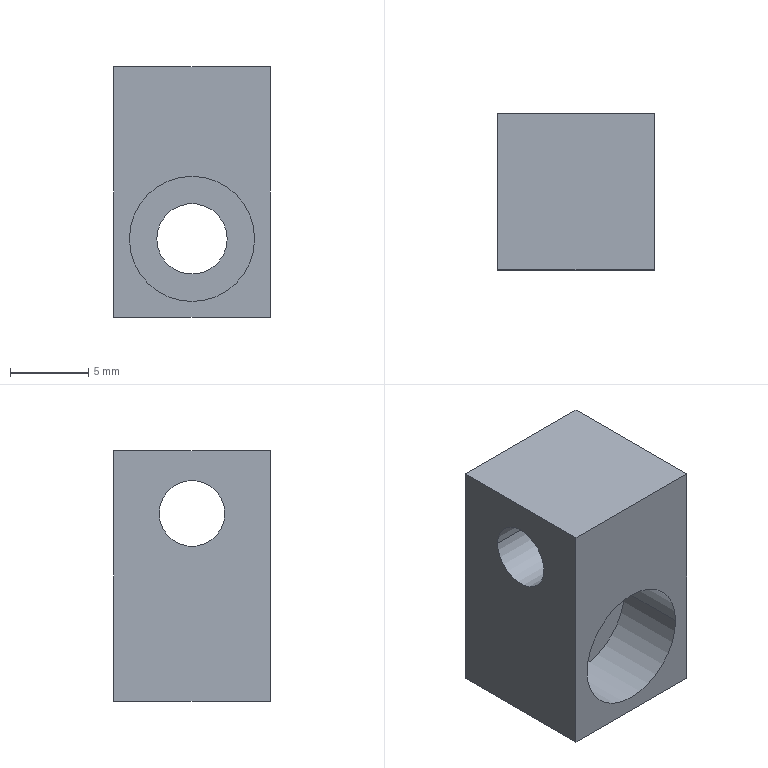Component | SolidWorks | 09HHHHHH8-2 | 1 solid | 13 faces | box 10 x 10 x 16 mm | volume 1144 mm3 | plane 7 | cylinder 6 | commonest cylinder face diameters 4.2 x2 8 x2 4.5 x2
build123d program:
from build123d import *

# Parameters (mm, degrees)
SKETCH1_W                                            = 10
SKETCH1_H                                            = 10
BOSS_EXTRUDE1_DEPTH                                  = 10
HOLE_SIZE_ACCORDING_TO_THE_TYPE_OF_HEXAG_D           = 4.5
HOLE_SIZE_ACCORDING_TO_THE_TYPE_OF_HEXAG_CBORE_D     = 8
HOLE_SIZE_ACCORDING_TO_THE_TYPE_OF_HEXAG_CBORE_DEPTH = 4.6
MOVE_FACE1_BY                                        = 6
M5_TAPPED_HOLE1_D                                    = 4.2
M5_TAPPED_HOLE1_DEPTH                                = 12.4
M5_TAPPED_HOLE1_TIP                                  = 1.262


with BuildPart() as part:
    # Sketch1 → Boss-Extrude1 (new body)
    with BuildSketch(Plane.XY):
        with Locations((610.359, -21.5)):
            Rectangle(SKETCH1_W, SKETCH1_H)
    extrude(amount=BOSS_EXTRUDE1_DEPTH)

    # Hole Size according to the type of hexag (through all)
    with Locations(Plane.XY.offset(10)):
        with Locations((610.359, -21.5)):
            CounterBoreHole(HOLE_SIZE_ACCORDING_TO_THE_TYPE_OF_HEXAG_D / 2, HOLE_SIZE_ACCORDING_TO_THE_TYPE_OF_HEXAG_CBORE_D / 2, HOLE_SIZE_ACCORDING_TO_THE_TYPE_OF_HEXAG_CBORE_DEPTH)

    # Move Face1: a face moved outward by 6.0
    extrude(part.faces().sort_by_distance((610.359, -16.5, 5))[0], amount=MOVE_FACE1_BY, dir=(0, 1, 0))

    # M5 Tapped Hole1
    with Locations(Plane(origin=(615.359, 0, 0), x_dir=(0, 0, -1), z_dir=(1, 0, 0))):
        with Locations((-5, -14.5)):
            Hole(M5_TAPPED_HOLE1_D / 2, depth=M5_TAPPED_HOLE1_DEPTH)
            with Locations((0, 0, -(M5_TAPPED_HOLE1_DEPTH + M5_TAPPED_HOLE1_TIP / 2))):  # 118° drill point
                Cone(0, M5_TAPPED_HOLE1_D / 2, M5_TAPPED_HOLE1_TIP, mode=Mode.SUBTRACT)


solid = part.part

# Placed as in the assembly
solid = solid.moved(Location((-1228.718, -304.383, 6.344), (90, 0, 0)))
STEP:
#1=COLOUR_RGB('',0.7922,0.8196,0.9333);
#2=FILL_AREA_STYLE_COLOUR('',#1);
#3=FILL_AREA_STYLE('',(#2));
#4=SURFACE_STYLE_FILL_AREA(#3);
#5=SURFACE_SIDE_STYLE('',(#4));
#6=SURFACE_STYLE_USAGE(.BOTH.,#5);
#7=PRESENTATION_STYLE_ASSIGNMENT((#6));
#8=CARTESIAN_POINT('',(-24.542,-12.263,-0.3211));
#9=VERTEX_POINT('',#8);
#10=CARTESIAN_POINT('',(-24.542,-12.098,-0.3211));
#11=VERTEX_POINT('',#10);
#12=CARTESIAN_POINT('',(-24.542,-12.18,-0.3211));
#13=DIRECTION('',(1.,0.,0.));
#14=DIRECTION('',(0.,1.,0.));
#15=AXIS2_PLACEMENT_3D('',#12,#13,#14);
#16=CIRCLE('',#15,0.08268);
#17=EDGE_CURVE('',#9,#11,#16,.T.);
#18=ORIENTED_EDGE('',*,*,#17,.F.);
#19=CARTESIAN_POINT('',(-24.148,-12.263,-0.3211));
#20=VERTEX_POINT('',#19);
#21=CARTESIAN_POINT('',(-24.148,-12.263,-0.3211));
#22=DIRECTION('',(1.,0.,0.));
#23=VECTOR('',#22,39.37);
#24=LINE('',#21,#23);
#25=EDGE_CURVE('',#9,#20,#24,.T.);
#26=ORIENTED_EDGE('',*,*,#25,.T.);
#27=CARTESIAN_POINT('',(-24.148,-12.098,-0.3211));
#28=VERTEX_POINT('',#27);
#29=CARTESIAN_POINT('',(-24.148,-12.18,-0.3211));
#30=DIRECTION('',(1.,0.,0.));
#31=DIRECTION('',(0.,1.,0.));
#32=AXIS2_PLACEMENT_3D('',#29,#30,#31);
#33=CIRCLE('',#32,0.08268);
#34=EDGE_CURVE('',#20,#28,#33,.T.);
#35=ORIENTED_EDGE('',*,*,#34,.T.);
#36=CARTESIAN_POINT('',(-24.148,-12.098,-0.3211));
#37=DIRECTION('',(1.,0.,0.));
#38=VECTOR('',#37,39.37);
#39=LINE('',#36,#38);
#40=EDGE_CURVE('',#11,#28,#39,.T.);
#41=ORIENTED_EDGE('',*,*,#40,.F.);
#42=EDGE_LOOP('',(#18,#26,#35,#41));
#43=FACE_OUTER_BOUND('',#42,.T.);
#44=CARTESIAN_POINT('',(-24.148,-12.18,-0.3211));
#45=DIRECTION('',(1.,0.,0.));
#46=DIRECTION('',(0.,1.,0.));
#47=AXIS2_PLACEMENT_3D('',#44,#45,#46);
#48=CYLINDRICAL_SURFACE('',#47,0.08268);
#49=ADVANCED_FACE('',(#43),#48,.F.);
#50=CARTESIAN_POINT('',(-24.502,-12.196,-0.5967));
#51=VERTEX_POINT('',#50);
#52=CARTESIAN_POINT('',(-24.187,-12.196,-0.5967));
#53=VERTEX_POINT('',#52);
#54=CARTESIAN_POINT('',(-24.345,-12.196,-0.5967));
#55=DIRECTION('',(0.,-1.,0.));
#56=DIRECTION('',(1.,0.,0.));
#57=AXIS2_PLACEMENT_3D('',#54,#55,#56);
#58=CIRCLE('',#57,0.1575);
#59=EDGE_CURVE('',#51,#53,#58,.T.);
#60=ORIENTED_EDGE('',*,*,#59,.F.);
#61=CARTESIAN_POINT('',(-24.502,-12.377,-0.5967));
#62=VERTEX_POINT('',#61);
#63=CARTESIAN_POINT('',(-24.502,-12.377,-0.5967));
#64=DIRECTION('',(0.,-1.,0.));
#65=VECTOR('',#64,39.37);
#66=LINE('',#63,#65);
#67=EDGE_CURVE('',#51,#62,#66,.T.);
#68=ORIENTED_EDGE('',*,*,#67,.T.);
#69=CARTESIAN_POINT('',(-24.187,-12.377,-0.5967));
#70=VERTEX_POINT('',#69);
#71=CARTESIAN_POINT('',(-24.345,-12.377,-0.5967));
#72=DIRECTION('',(0.,-1.,0.));
#73=DIRECTION('',(1.,0.,0.));
#74=AXIS2_PLACEMENT_3D('',#71,#72,#73);
#75=CIRCLE('',#74,0.1575);
#76=EDGE_CURVE('',#62,#70,#75,.T.);
#77=ORIENTED_EDGE('',*,*,#76,.T.);
#78=CARTESIAN_POINT('',(-24.187,-12.377,-0.5967));
#79=DIRECTION('',(0.,-1.,0.));
#80=VECTOR('',#79,39.37);
#81=LINE('',#78,#80);
#82=EDGE_CURVE('',#53,#70,#81,.T.);
#83=ORIENTED_EDGE('',*,*,#82,.F.);
#84=EDGE_LOOP('',(#60,#68,#77,#83));
#85=FACE_OUTER_BOUND('',#84,.T.);
#86=CARTESIAN_POINT('',(-24.345,-12.377,-0.5967));
#87=DIRECTION('',(0.,-1.,0.));
#88=DIRECTION('',(1.,0.,0.));
#89=AXIS2_PLACEMENT_3D('',#86,#87,#88);
#90=CYLINDRICAL_SURFACE('',#89,0.1575);
#91=ADVANCED_FACE('',(#85),#90,.F.);
#92=CARTESIAN_POINT('',(-24.433,-11.984,-0.5967));
#93=VERTEX_POINT('',#92);
#94=CARTESIAN_POINT('',(-24.256,-11.984,-0.5967));
#95=VERTEX_POINT('',#94);
#96=CARTESIAN_POINT('',(-24.345,-11.984,-0.5967));
#97=DIRECTION('',(0.,-1.,0.));
#98=DIRECTION('',(1.,0.,0.));
#99=AXIS2_PLACEMENT_3D('',#96,#97,#98);
#100=CIRCLE('',#99,0.08858);
#101=EDGE_CURVE('',#93,#95,#100,.T.);
#102=ORIENTED_EDGE('',*,*,#101,.F.);
#103=CARTESIAN_POINT('',(-24.433,-12.196,-0.5967));
#104=VERTEX_POINT('',#103);
#105=CARTESIAN_POINT('',(-24.433,-12.377,-0.5967));
#106=DIRECTION('',(0.,-1.,0.));
#107=VECTOR('',#106,39.37);
#108=LINE('',#105,#107);
#109=EDGE_CURVE('',#93,#104,#108,.T.);
#110=ORIENTED_EDGE('',*,*,#109,.T.);
#111=CARTESIAN_POINT('',(-24.256,-12.196,-0.5967));
#112=VERTEX_POINT('',#111);
#113=CARTESIAN_POINT('',(-24.345,-12.196,-0.5967));
#114=DIRECTION('',(0.,-1.,0.));
#115=DIRECTION('',(1.,0.,0.));
#116=AXIS2_PLACEMENT_3D('',#113,#114,#115);
#117=CIRCLE('',#116,0.08858);
#118=EDGE_CURVE('',#104,#112,#117,.T.);
#119=ORIENTED_EDGE('',*,*,#118,.T.);
#120=CARTESIAN_POINT('',(-24.256,-12.377,-0.5967));
#121=DIRECTION('',(0.,-1.,0.));
#122=VECTOR('',#121,39.37);
#123=LINE('',#120,#122);
#124=EDGE_CURVE('',#95,#112,#123,.T.);
#125=ORIENTED_EDGE('',*,*,#124,.F.);
#126=EDGE_LOOP('',(#102,#110,#119,#125));
#127=FACE_OUTER_BOUND('',#126,.T.);
#128=CARTESIAN_POINT('',(-24.345,-12.377,-0.5967));
#129=DIRECTION('',(0.,-1.,0.));
#130=DIRECTION('',(1.,0.,0.));
#131=AXIS2_PLACEMENT_3D('',#128,#129,#130);
#132=CYLINDRICAL_SURFACE('',#131,0.08858);
#133=ADVANCED_FACE('',(#127),#132,.F.);
#134=CARTESIAN_POINT('',(-24.542,-12.18,-0.3211));
#135=DIRECTION('',(1.,0.,0.));
#136=DIRECTION('',(0.,1.,0.));
#137=AXIS2_PLACEMENT_3D('',#134,#135,#136);
#138=CIRCLE('',#137,0.08268);
#139=EDGE_CURVE('',#11,#9,#138,.T.);
#140=ORIENTED_EDGE('',*,*,#139,.T.);
#141=ORIENTED_EDGE('',*,*,#17,.T.);
#142=EDGE_LOOP('',(#140,#141));
#143=FACE_BOUND('',#142,.T.);
#144=CARTESIAN_POINT('',(-24.542,-11.984,-0.1636));
#145=VERTEX_POINT('',#144);
#146=CARTESIAN_POINT('',(-24.542,-11.984,-0.7936));
#147=VERTEX_POINT('',#146);
#148=CARTESIAN_POINT('',(-24.542,-11.984,-0.3999));
#149=DIRECTION('',(0.,0.,-1.));
#150=VECTOR('',#149,39.37);
#151=LINE('',#148,#150);
#152=EDGE_CURVE('',#145,#147,#151,.T.);
#153=ORIENTED_EDGE('',*,*,#152,.T.);
#154=CARTESIAN_POINT('',(-24.542,-12.377,-0.7936));
#155=VERTEX_POINT('',#154);
#156=CARTESIAN_POINT('',(-24.542,-12.377,-0.7936));
#157=DIRECTION('',(0.,1.,0.));
#158=VECTOR('',#157,39.37);
#159=LINE('',#156,#158);
#160=EDGE_CURVE('',#155,#147,#159,.T.);
#161=ORIENTED_EDGE('',*,*,#160,.F.);
#162=CARTESIAN_POINT('',(-24.542,-12.377,-0.1636));
#163=VERTEX_POINT('',#162);
#164=CARTESIAN_POINT('',(-24.542,-12.377,-0.3999));
#165=DIRECTION('',(0.,0.,-1.));
#166=VECTOR('',#165,39.37);
#167=LINE('',#164,#166);
#168=EDGE_CURVE('',#163,#155,#167,.T.);
#169=ORIENTED_EDGE('',*,*,#168,.F.);
#170=CARTESIAN_POINT('',(-24.542,-12.377,-0.1636));
#171=DIRECTION('',(0.,1.,0.));
#172=VECTOR('',#171,39.37);
#173=LINE('',#170,#172);
#174=EDGE_CURVE('',#163,#145,#173,.T.);
#175=ORIENTED_EDGE('',*,*,#174,.T.);
#176=EDGE_LOOP('',(#153,#161,#169,#175));
#177=FACE_OUTER_BOUND('',#176,.T.);
#178=CARTESIAN_POINT('',(-24.542,-12.377,-0.3999));
#179=DIRECTION('',(1.,0.,0.));
#180=DIRECTION('',(0.,1.,0.));
#181=AXIS2_PLACEMENT_3D('',#178,#179,#180);
#182=PLANE('',#181);
#183=ADVANCED_FACE('',(#143,#177),#182,.F.);
#184=CARTESIAN_POINT('',(-24.148,-11.984,-0.7936));
#185=VERTEX_POINT('',#184);
#186=CARTESIAN_POINT('',(-24.542,-11.984,-0.7936));
#187=DIRECTION('',(1.,0.,0.));
#188=VECTOR('',#187,39.37);
#189=LINE('',#186,#188);
#190=EDGE_CURVE('',#147,#185,#189,.T.);
#191=ORIENTED_EDGE('',*,*,#190,.T.);
#192=CARTESIAN_POINT('',(-24.148,-12.377,-0.7936));
#193=VERTEX_POINT('',#192);
#194=CARTESIAN_POINT('',(-24.148,-12.377,-0.7936));
#195=DIRECTION('',(0.,1.,0.));
#196=VECTOR('',#195,39.37);
#197=LINE('',#194,#196);
#198=EDGE_CURVE('',#193,#185,#197,.T.);
#199=ORIENTED_EDGE('',*,*,#198,.F.);
#200=CARTESIAN_POINT('',(-24.542,-12.377,-0.7936));
#201=DIRECTION('',(1.,0.,0.));
#202=VECTOR('',#201,39.37);
#203=LINE('',#200,#202);
#204=EDGE_CURVE('',#155,#193,#203,.T.);
#205=ORIENTED_EDGE('',*,*,#204,.F.);
#206=ORIENTED_EDGE('',*,*,#160,.T.);
#207=EDGE_LOOP('',(#191,#199,#205,#206));
#208=FACE_OUTER_BOUND('',#207,.T.);
#209=CARTESIAN_POINT('',(-24.542,-12.377,-0.7936));
#210=DIRECTION('',(-0.,0.,1.));
#211=DIRECTION('',(0.,-1.,0.));
#212=AXIS2_PLACEMENT_3D('',#209,#210,#211);
#213=PLANE('',#212);
#214=ADVANCED_FACE('',(#208),#213,.F.);
#215=CARTESIAN_POINT('',(-24.148,-12.18,-0.3211));
#216=DIRECTION('',(1.,0.,0.));
#217=DIRECTION('',(0.,1.,0.));
#218=AXIS2_PLACEMENT_3D('',#215,#216,#217);
#219=CIRCLE('',#218,0.08268);
#220=EDGE_CURVE('',#28,#20,#219,.T.);
#221=ORIENTED_EDGE('',*,*,#220,.F.);
#222=ORIENTED_EDGE('',*,*,#34,.F.);
#223=EDGE_LOOP('',(#221,#222));
#224=FACE_BOUND('',#223,.T.);
#225=CARTESIAN_POINT('',(-24.148,-11.984,-0.1636));
#226=VERTEX_POINT('',#225);
#227=CARTESIAN_POINT('',(-24.148,-11.984,-0.3999));
#228=DIRECTION('',(-0.,0.,1.));
#229=VECTOR('',#228,39.37);
#230=LINE('',#227,#229);
#231=EDGE_CURVE('',#185,#226,#230,.T.);
#232=ORIENTED_EDGE('',*,*,#231,.T.);
#233=CARTESIAN_POINT('',(-24.148,-12.377,-0.1636));
#234=VERTEX_POINT('',#233);
#235=CARTESIAN_POINT('',(-24.148,-12.377,-0.1636));
#236=DIRECTION('',(0.,1.,0.));
#237=VECTOR('',#236,39.37);
#238=LINE('',#235,#237);
#239=EDGE_CURVE('',#234,#226,#238,.T.);
#240=ORIENTED_EDGE('',*,*,#239,.F.);
#241=CARTESIAN_POINT('',(-24.148,-12.377,-0.3999));
#242=DIRECTION('',(-0.,0.,1.));
#243=VECTOR('',#242,39.37);
#244=LINE('',#241,#243);
#245=EDGE_CURVE('',#193,#234,#244,.T.);
#246=ORIENTED_EDGE('',*,*,#245,.F.);
#247=ORIENTED_EDGE('',*,*,#198,.T.);
#248=EDGE_LOOP('',(#232,#240,#246,#247));
#249=FACE_OUTER_BOUND('',#248,.T.);
#250=CARTESIAN_POINT('',(-24.148,-12.377,-0.3999));
#251=DIRECTION('',(-1.,0.,-0.));
#252=DIRECTION('',(0.,-1.,0.));
#253=AXIS2_PLACEMENT_3D('',#250,#251,#252);
#254=PLANE('',#253);
#255=ADVANCED_FACE('',(#224,#249),#254,.F.);
#256=CARTESIAN_POINT('',(-24.542,-11.984,-0.1636));
#257=DIRECTION('',(-1.,0.,-0.));
#258=VECTOR('',#257,39.37);
#259=LINE('',#256,#258);
#260=EDGE_CURVE('',#226,#145,#259,.T.);
#261=ORIENTED_EDGE('',*,*,#260,.T.);
#262=ORIENTED_EDGE('',*,*,#174,.F.);
#263=CARTESIAN_POINT('',(-24.542,-12.377,-0.1636));
#264=DIRECTION('',(-1.,0.,-0.));
#265=VECTOR('',#264,39.37);
#266=LINE('',#263,#265);
#267=EDGE_CURVE('',#234,#163,#266,.T.);
#268=ORIENTED_EDGE('',*,*,#267,.F.);
#269=ORIENTED_EDGE('',*,*,#239,.T.);
#270=EDGE_LOOP('',(#261,#262,#268,#269));
#271=FACE_OUTER_BOUND('',#270,.T.);
#272=CARTESIAN_POINT('',(-24.542,-12.377,-0.1636));
#273=DIRECTION('',(0.,0.,-1.));
#274=DIRECTION('',(0.,1.,0.));
#275=AXIS2_PLACEMENT_3D('',#272,#273,#274);
#276=PLANE('',#275);
#277=ADVANCED_FACE('',(#271),#276,.F.);
#278=CARTESIAN_POINT('',(-24.345,-12.377,-0.5967));
#279=DIRECTION('',(0.,-1.,0.));
#280=DIRECTION('',(1.,0.,0.));
#281=AXIS2_PLACEMENT_3D('',#278,#279,#280);
#282=CIRCLE('',#281,0.1575);
#283=EDGE_CURVE('',#70,#62,#282,.T.);
#284=ORIENTED_EDGE('',*,*,#283,.F.);
#285=ORIENTED_EDGE('',*,*,#76,.F.);
#286=EDGE_LOOP('',(#284,#285));
#287=FACE_BOUND('',#286,.T.);
#288=ORIENTED_EDGE('',*,*,#168,.T.);
#289=ORIENTED_EDGE('',*,*,#204,.T.);
#290=ORIENTED_EDGE('',*,*,#245,.T.);
#291=ORIENTED_EDGE('',*,*,#267,.T.);
#292=EDGE_LOOP('',(#288,#289,#290,#291));
#293=FACE_OUTER_BOUND('',#292,.T.);
#294=CARTESIAN_POINT('',(-48.375,-12.377,0.2498));
#295=DIRECTION('',(0.,-1.,0.));
#296=DIRECTION('',(1.,0.,0.));
#297=AXIS2_PLACEMENT_3D('',#294,#295,#296);
#298=PLANE('',#297);
#299=ADVANCED_FACE('',(#287,#293),#298,.T.);
#300=CARTESIAN_POINT('',(-24.345,-11.984,-0.5967));
#301=DIRECTION('',(0.,-1.,0.));
#302=DIRECTION('',(1.,0.,0.));
#303=AXIS2_PLACEMENT_3D('',#300,#301,#302);
#304=CIRCLE('',#303,0.08858);
#305=EDGE_CURVE('',#95,#93,#304,.T.);
#306=ORIENTED_EDGE('',*,*,#305,.T.);
#307=ORIENTED_EDGE('',*,*,#101,.T.);
#308=EDGE_LOOP('',(#306,#307));
#309=FACE_BOUND('',#308,.T.);
#310=ORIENTED_EDGE('',*,*,#152,.F.);
#311=ORIENTED_EDGE('',*,*,#260,.F.);
#312=ORIENTED_EDGE('',*,*,#231,.F.);
#313=ORIENTED_EDGE('',*,*,#190,.F.);
#314=EDGE_LOOP('',(#310,#311,#312,#313));
#315=FACE_OUTER_BOUND('',#314,.T.);
#316=CARTESIAN_POINT('',(-48.375,-11.984,0.2498));
#317=DIRECTION('',(0.,-1.,0.));
#318=DIRECTION('',(1.,0.,0.));
#319=AXIS2_PLACEMENT_3D('',#316,#317,#318);
#320=PLANE('',#319);
#321=ADVANCED_FACE('',(#309,#315),#320,.F.);
#322=ORIENTED_EDGE('',*,*,#109,.F.);
#323=ORIENTED_EDGE('',*,*,#305,.F.);
#324=ORIENTED_EDGE('',*,*,#124,.T.);
#325=CARTESIAN_POINT('',(-24.345,-12.196,-0.5967));
#326=DIRECTION('',(0.,-1.,0.));
#327=DIRECTION('',(1.,0.,0.));
#328=AXIS2_PLACEMENT_3D('',#325,#326,#327);
#329=CIRCLE('',#328,0.08858);
#330=EDGE_CURVE('',#112,#104,#329,.T.);
#331=ORIENTED_EDGE('',*,*,#330,.T.);
#332=EDGE_LOOP('',(#322,#323,#324,#331));
#333=FACE_OUTER_BOUND('',#332,.T.);
#334=CARTESIAN_POINT('',(-24.345,-12.377,-0.5967));
#335=DIRECTION('',(0.,-1.,0.));
#336=DIRECTION('',(1.,0.,0.));
#337=AXIS2_PLACEMENT_3D('',#334,#335,#336);
#338=CYLINDRICAL_SURFACE('',#337,0.08858);
#339=ADVANCED_FACE('',(#333),#338,.F.);
#340=ORIENTED_EDGE('',*,*,#330,.F.);
#341=ORIENTED_EDGE('',*,*,#118,.F.);
#342=EDGE_LOOP('',(#340,#341));
#343=FACE_BOUND('',#342,.T.);
#344=CARTESIAN_POINT('',(-24.345,-12.196,-0.5967));
#345=DIRECTION('',(0.,-1.,0.));
#346=DIRECTION('',(1.,0.,0.));
#347=AXIS2_PLACEMENT_3D('',#344,#345,#346);
#348=CIRCLE('',#347,0.1575);
#349=EDGE_CURVE('',#53,#51,#348,.T.);
#350=ORIENTED_EDGE('',*,*,#349,.T.);
#351=ORIENTED_EDGE('',*,*,#59,.T.);
#352=EDGE_LOOP('',(#350,#351));
#353=FACE_OUTER_BOUND('',#352,.T.);
#354=CARTESIAN_POINT('',(-24.256,-12.196,-0.5967));
#355=DIRECTION('',(0.,1.,0.));
#356=DIRECTION('',(-1.,0.,-0.));
#357=AXIS2_PLACEMENT_3D('',#354,#355,#356);
#358=PLANE('',#357);
#359=ADVANCED_FACE('',(#343,#353),#358,.F.);
#360=ORIENTED_EDGE('',*,*,#67,.F.);
#361=ORIENTED_EDGE('',*,*,#349,.F.);
#362=ORIENTED_EDGE('',*,*,#82,.T.);
#363=ORIENTED_EDGE('',*,*,#283,.T.);
#364=EDGE_LOOP('',(#360,#361,#362,#363));
#365=FACE_OUTER_BOUND('',#364,.T.);
#366=CARTESIAN_POINT('',(-24.345,-12.377,-0.5967));
#367=DIRECTION('',(0.,-1.,0.));
#368=DIRECTION('',(1.,0.,0.));
#369=AXIS2_PLACEMENT_3D('',#366,#367,#368);
#370=CYLINDRICAL_SURFACE('',#369,0.1575);
#371=ADVANCED_FACE('',(#365),#370,.F.);
#372=ORIENTED_EDGE('',*,*,#25,.F.);
#373=ORIENTED_EDGE('',*,*,#139,.F.);
#374=ORIENTED_EDGE('',*,*,#40,.T.);
#375=ORIENTED_EDGE('',*,*,#220,.T.);
#376=EDGE_LOOP('',(#372,#373,#374,#375));
#377=FACE_OUTER_BOUND('',#376,.T.);
#378=CARTESIAN_POINT('',(-24.148,-12.18,-0.3211));
#379=DIRECTION('',(1.,0.,0.));
#380=DIRECTION('',(0.,1.,0.));
#381=AXIS2_PLACEMENT_3D('',#378,#379,#380);
#382=CYLINDRICAL_SURFACE('',#381,0.08268);
#383=ADVANCED_FACE('',(#377),#382,.F.);
#384=CLOSED_SHELL('',(#49,#91,#133,#183,#214,#255,#277,#299,#321,#339,#359,#371,#383));
#385=MANIFOLD_SOLID_BREP('',#384);
#386=STYLED_ITEM('',(#7),#385);
#387=(LENGTH_UNIT()NAMED_UNIT(*)SI_UNIT($,.METRE.));
#388=LENGTH_MEASURE_WITH_UNIT(LENGTH_MEASURE(0.0254),#387);
#389=DIMENSIONAL_EXPONENTS(1.,0.,0.,0.,0.,0.,0.);
#390=(CONVERSION_BASED_UNIT('',#388)LENGTH_UNIT()NAMED_UNIT(#389));
#391=UNCERTAINTY_MEASURE_WITH_UNIT(LENGTH_MEASURE(0.00001),#390,'','');
#392=(NAMED_UNIT(*)PLANE_ANGLE_UNIT()SI_UNIT($,.RADIAN.));
#393=(NAMED_UNIT(*)SI_UNIT($,.STERADIAN.)SOLID_ANGLE_UNIT());
#394=(GEOMETRIC_REPRESENTATION_CONTEXT(3)GLOBAL_UNCERTAINTY_ASSIGNED_CONTEXT((#391))GLOBAL_UNIT_ASSIGNED_CONTEXT((#390,#392,#393))REPRESENTATION_CONTEXT('',''));
#395=MECHANICAL_DESIGN_GEOMETRIC_PRESENTATION_REPRESENTATION('',(#386),#394);
#396=CARTESIAN_POINT('',(0.,0.,0.));
#397=DIRECTION('',(0.,0.,1.));
#398=DIRECTION('',(1.,0.,0.));
#399=AXIS2_PLACEMENT_3D('',#396,#397,#398);
#400=(LENGTH_UNIT()NAMED_UNIT(*)SI_UNIT($,.METRE.));
#401=LENGTH_MEASURE_WITH_UNIT(LENGTH_MEASURE(0.0254),#400);
#402=DIMENSIONAL_EXPONENTS(1.,0.,0.,0.,0.,0.,0.);
#403=(CONVERSION_BASED_UNIT('',#401)LENGTH_UNIT()NAMED_UNIT(#402));
#404=UNCERTAINTY_MEASURE_WITH_UNIT(LENGTH_MEASURE(0.00001),#403,'','');
#405=(NAMED_UNIT(*)PLANE_ANGLE_UNIT()SI_UNIT($,.RADIAN.));
#406=(NAMED_UNIT(*)SI_UNIT($,.STERADIAN.)SOLID_ANGLE_UNIT());
#407=(GEOMETRIC_REPRESENTATION_CONTEXT(3)GLOBAL_UNCERTAINTY_ASSIGNED_CONTEXT((#404))GLOBAL_UNIT_ASSIGNED_CONTEXT((#403,#405,#406))REPRESENTATION_CONTEXT('',''));
#408=ADVANCED_BREP_SHAPE_REPRESENTATION('',(#385,#399),#407);
#409=PRESENTATION_LAYER_ASSIGNMENT('','',(#386));